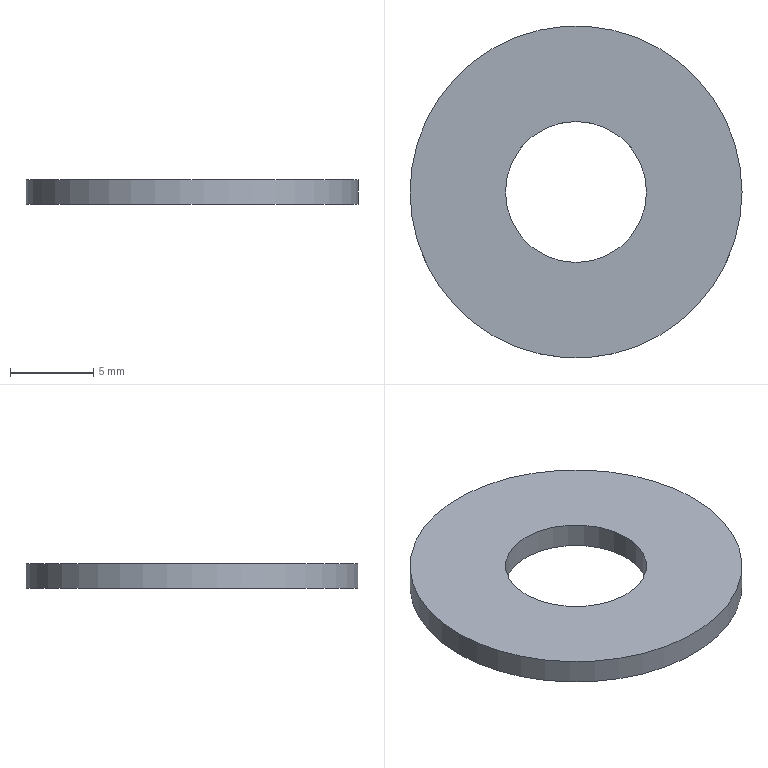Component | NX | WASHER | 1 solid | 4 faces | box 20 x 20 x 1.5 mm | volume 386 mm3 | cylinder 2 | plane 2 | commonest cylinder face diameters 20 x1 8.5 x1
STEP:
#1=CARTESIAN_POINT('',(0.,0.,0.));
#2=DIRECTION('',(0.,0.,1.));
#3=DIRECTION('',(1.,0.,0.));
#4=AXIS2_PLACEMENT_3D('',#1,#2,#3);
#5=CARTESIAN_POINT('',(36.422,91.456,-21.));
#6=VERTEX_POINT('',#5);
#7=CARTESIAN_POINT('',(26.422,91.456,-21.));
#8=DIRECTION('',(0.,0.,-1.));
#9=DIRECTION('',(1.,0.,0.));
#10=AXIS2_PLACEMENT_3D('',#7,#8,#9);
#11=CIRCLE('',#10,10.);
#12=CARTESIAN_POINT('',(26.422,91.456,-21.));
#13=DIRECTION('',(0.,0.,1.));
#14=DIRECTION('',(-1.,0.,0.));
#15=AXIS2_PLACEMENT_3D('',#12,#13,#14);
#16=CYLINDRICAL_SURFACE('',#15,10.);
#17=CARTESIAN_POINT('',(9.425,0.));
#18=DIRECTION('',(-1.,0.));
#19=VECTOR('',#18,1.);
#20=LINE('',#17,#19);
#21=(GEOMETRIC_REPRESENTATION_CONTEXT(2)PARAMETRIC_REPRESENTATION_CONTEXT()REPRESENTATION_CONTEXT('',''));
#22=DEFINITIONAL_REPRESENTATION('',(#20),#21);
#23=PCURVE('',#16,#22);
#24=CARTESIAN_POINT('',(26.422,91.456,-21.));
#25=DIRECTION('',(0.,0.,-1.));
#26=DIRECTION('',(1.,0.,0.));
#27=AXIS2_PLACEMENT_3D('',#24,#25,#26);
#28=PLANE('',#27);
#29=CARTESIAN_POINT('',(0.,0.));
#30=DIRECTION('',(1.,0.));
#31=AXIS2_PLACEMENT_2D('',#29,#30);
#32=CIRCLE('',#31,10.);
#33=(GEOMETRIC_REPRESENTATION_CONTEXT(2)PARAMETRIC_REPRESENTATION_CONTEXT()REPRESENTATION_CONTEXT('',''));
#34=DEFINITIONAL_REPRESENTATION('',(#32),#33);
#35=PCURVE('',#28,#34);
#36=SURFACE_CURVE('',#11,(#23,#35),.PCURVE_S1.);
#37=EDGE_CURVE('',#6,#6,#36,.T.);
#38=ORIENTED_EDGE('',*,*,#37,.F.);
#39=CARTESIAN_POINT('',(36.422,91.456,-19.5));
#40=VERTEX_POINT('',#39);
#41=CARTESIAN_POINT('',(36.422,91.456,-21.));
#42=CARTESIAN_POINT('',(36.422,91.456,-19.5));
#43=B_SPLINE_CURVE_WITH_KNOTS('',1,(#41,#42),.UNSPECIFIED.,.F.,.F.,(2,2),(0.,1.5),.PIECEWISE_BEZIER_KNOTS.);
#44=CARTESIAN_POINT('',(9.425,0.));
#45=DIRECTION('',(0.,1.));
#46=VECTOR('',#45,1.);
#47=LINE('',#44,#46);
#48=(GEOMETRIC_REPRESENTATION_CONTEXT(2)PARAMETRIC_REPRESENTATION_CONTEXT()REPRESENTATION_CONTEXT('',''));
#49=DEFINITIONAL_REPRESENTATION('',(#47),#48);
#50=PCURVE('',#16,#49);
#51=CARTESIAN_POINT('',(3.142,0.));
#52=DIRECTION('',(0.,1.));
#53=VECTOR('',#52,1.);
#54=LINE('',#51,#53);
#55=(GEOMETRIC_REPRESENTATION_CONTEXT(2)PARAMETRIC_REPRESENTATION_CONTEXT()REPRESENTATION_CONTEXT('',''));
#56=DEFINITIONAL_REPRESENTATION('',(#54),#55);
#57=PCURVE('',#16,#56);
#58=SEAM_CURVE('',#43,(#50,#57),.PCURVE_S1.);
#59=EDGE_CURVE('',#6,#40,#58,.T.);
#60=ORIENTED_EDGE('',*,*,#59,.T.);
#61=CARTESIAN_POINT('',(26.422,91.456,-19.5));
#62=DIRECTION('',(0.,0.,-1.));
#63=DIRECTION('',(1.,0.,0.));
#64=AXIS2_PLACEMENT_3D('',#61,#62,#63);
#65=CIRCLE('',#64,10.);
#66=CARTESIAN_POINT('',(9.425,1.5));
#67=DIRECTION('',(-1.,0.));
#68=VECTOR('',#67,1.);
#69=LINE('',#66,#68);
#70=(GEOMETRIC_REPRESENTATION_CONTEXT(2)PARAMETRIC_REPRESENTATION_CONTEXT()REPRESENTATION_CONTEXT('',''));
#71=DEFINITIONAL_REPRESENTATION('',(#69),#70);
#72=PCURVE('',#16,#71);
#73=CARTESIAN_POINT('',(26.422,91.456,-19.5));
#74=DIRECTION('',(0.,0.,-1.));
#75=DIRECTION('',(1.,0.,0.));
#76=AXIS2_PLACEMENT_3D('',#73,#74,#75);
#77=PLANE('',#76);
#78=CARTESIAN_POINT('',(0.,0.));
#79=DIRECTION('',(1.,0.));
#80=AXIS2_PLACEMENT_2D('',#78,#79);
#81=CIRCLE('',#80,10.);
#82=(GEOMETRIC_REPRESENTATION_CONTEXT(2)PARAMETRIC_REPRESENTATION_CONTEXT()REPRESENTATION_CONTEXT('',''));
#83=DEFINITIONAL_REPRESENTATION('',(#81),#82);
#84=PCURVE('',#77,#83);
#85=SURFACE_CURVE('',#65,(#72,#84),.PCURVE_S1.);
#86=EDGE_CURVE('',#40,#40,#85,.T.);
#87=ORIENTED_EDGE('',*,*,#86,.T.);
#88=ORIENTED_EDGE('',*,*,#59,.F.);
#89=EDGE_LOOP('',(#38,#60,#87,#88));
#90=FACE_BOUND('',#89,.T.);
#91=ADVANCED_FACE('',(#90),#16,.T.);
#92=CARTESIAN_POINT('',(30.672,91.456,-21.));
#93=VERTEX_POINT('',#92);
#94=CARTESIAN_POINT('',(26.422,91.456,-21.));
#95=DIRECTION('',(0.,0.,-1.));
#96=DIRECTION('',(1.,0.,0.));
#97=AXIS2_PLACEMENT_3D('',#94,#95,#96);
#98=CIRCLE('',#97,4.25);
#99=CARTESIAN_POINT('',(26.422,91.456,-21.));
#100=DIRECTION('',(0.,0.,1.));
#101=DIRECTION('',(-1.,0.,0.));
#102=AXIS2_PLACEMENT_3D('',#99,#100,#101);
#103=CYLINDRICAL_SURFACE('',#102,4.25);
#104=CARTESIAN_POINT('',(9.425,0.));
#105=DIRECTION('',(-1.,0.));
#106=VECTOR('',#105,1.);
#107=LINE('',#104,#106);
#108=(GEOMETRIC_REPRESENTATION_CONTEXT(2)PARAMETRIC_REPRESENTATION_CONTEXT()REPRESENTATION_CONTEXT('',''));
#109=DEFINITIONAL_REPRESENTATION('',(#107),#108);
#110=PCURVE('',#103,#109);
#111=CARTESIAN_POINT('',(0.,0.));
#112=DIRECTION('',(1.,0.));
#113=AXIS2_PLACEMENT_2D('',#111,#112);
#114=CIRCLE('',#113,4.25);
#115=(GEOMETRIC_REPRESENTATION_CONTEXT(2)PARAMETRIC_REPRESENTATION_CONTEXT()REPRESENTATION_CONTEXT('',''));
#116=DEFINITIONAL_REPRESENTATION('',(#114),#115);
#117=PCURVE('',#28,#116);
#118=SURFACE_CURVE('',#98,(#110,#117),.PCURVE_S1.);
#119=EDGE_CURVE('',#93,#93,#118,.T.);
#120=ORIENTED_EDGE('',*,*,#119,.F.);
#121=CARTESIAN_POINT('',(30.672,91.456,-19.5));
#122=VERTEX_POINT('',#121);
#123=CARTESIAN_POINT('',(30.672,91.456,-21.));
#124=CARTESIAN_POINT('',(30.672,91.456,-19.5));
#125=B_SPLINE_CURVE_WITH_KNOTS('',1,(#123,#124),.UNSPECIFIED.,.F.,.F.,(2,2),(0.,1.5),.PIECEWISE_BEZIER_KNOTS.);
#126=CARTESIAN_POINT('',(9.425,0.));
#127=DIRECTION('',(0.,1.));
#128=VECTOR('',#127,1.);
#129=LINE('',#126,#128);
#130=(GEOMETRIC_REPRESENTATION_CONTEXT(2)PARAMETRIC_REPRESENTATION_CONTEXT()REPRESENTATION_CONTEXT('',''));
#131=DEFINITIONAL_REPRESENTATION('',(#129),#130);
#132=PCURVE('',#103,#131);
#133=CARTESIAN_POINT('',(3.142,0.));
#134=DIRECTION('',(0.,1.));
#135=VECTOR('',#134,1.);
#136=LINE('',#133,#135);
#137=(GEOMETRIC_REPRESENTATION_CONTEXT(2)PARAMETRIC_REPRESENTATION_CONTEXT()REPRESENTATION_CONTEXT('',''));
#138=DEFINITIONAL_REPRESENTATION('',(#136),#137);
#139=PCURVE('',#103,#138);
#140=SEAM_CURVE('',#125,(#132,#139),.PCURVE_S1.);
#141=EDGE_CURVE('',#93,#122,#140,.T.);
#142=ORIENTED_EDGE('',*,*,#141,.T.);
#143=CARTESIAN_POINT('',(26.422,91.456,-19.5));
#144=DIRECTION('',(0.,0.,-1.));
#145=DIRECTION('',(1.,0.,0.));
#146=AXIS2_PLACEMENT_3D('',#143,#144,#145);
#147=CIRCLE('',#146,4.25);
#148=CARTESIAN_POINT('',(9.425,1.5));
#149=DIRECTION('',(-1.,0.));
#150=VECTOR('',#149,1.);
#151=LINE('',#148,#150);
#152=(GEOMETRIC_REPRESENTATION_CONTEXT(2)PARAMETRIC_REPRESENTATION_CONTEXT()REPRESENTATION_CONTEXT('',''));
#153=DEFINITIONAL_REPRESENTATION('',(#151),#152);
#154=PCURVE('',#103,#153);
#155=CARTESIAN_POINT('',(0.,0.));
#156=DIRECTION('',(1.,0.));
#157=AXIS2_PLACEMENT_2D('',#155,#156);
#158=CIRCLE('',#157,4.25);
#159=(GEOMETRIC_REPRESENTATION_CONTEXT(2)PARAMETRIC_REPRESENTATION_CONTEXT()REPRESENTATION_CONTEXT('',''));
#160=DEFINITIONAL_REPRESENTATION('',(#158),#159);
#161=PCURVE('',#77,#160);
#162=SURFACE_CURVE('',#147,(#154,#161),.PCURVE_S1.);
#163=EDGE_CURVE('',#122,#122,#162,.T.);
#164=ORIENTED_EDGE('',*,*,#163,.T.);
#165=ORIENTED_EDGE('',*,*,#141,.F.);
#166=EDGE_LOOP('',(#120,#142,#164,#165));
#167=FACE_BOUND('',#166,.F.);
#168=ADVANCED_FACE('',(#167),#103,.F.);
#169=ORIENTED_EDGE('',*,*,#37,.T.);
#170=EDGE_LOOP('',(#169));
#171=FACE_BOUND('',#170,.T.);
#172=ORIENTED_EDGE('',*,*,#119,.F.);
#173=EDGE_LOOP('',(#172));
#174=FACE_BOUND('',#173,.T.);
#175=ADVANCED_FACE('',(#171,#174),#28,.T.);
#176=ORIENTED_EDGE('',*,*,#86,.F.);
#177=EDGE_LOOP('',(#176));
#178=FACE_BOUND('',#177,.T.);
#179=ORIENTED_EDGE('',*,*,#163,.T.);
#180=EDGE_LOOP('',(#179));
#181=FACE_BOUND('',#180,.T.);
#182=ADVANCED_FACE('',(#178,#181),#77,.F.);
#183=CLOSED_SHELL('',(#91,#168,#175,#182));
#184=MANIFOLD_SOLID_BREP('',#183);
#185=(LENGTH_UNIT()NAMED_UNIT(*)SI_UNIT(.MILLI.,.METRE.));
#186=UNCERTAINTY_MEASURE_WITH_UNIT(LENGTH_MEASURE(0.00001),#185,'','');
#187=(NAMED_UNIT(*)PLANE_ANGLE_UNIT()SI_UNIT($,.RADIAN.));
#188=(NAMED_UNIT(*)SI_UNIT($,.STERADIAN.)SOLID_ANGLE_UNIT());
#189=(GEOMETRIC_REPRESENTATION_CONTEXT(3)GLOBAL_UNCERTAINTY_ASSIGNED_CONTEXT((#186))GLOBAL_UNIT_ASSIGNED_CONTEXT((#185,#187,#188))REPRESENTATION_CONTEXT('',''));
#190=ADVANCED_BREP_SHAPE_REPRESENTATION('',(#4,#184),#189);